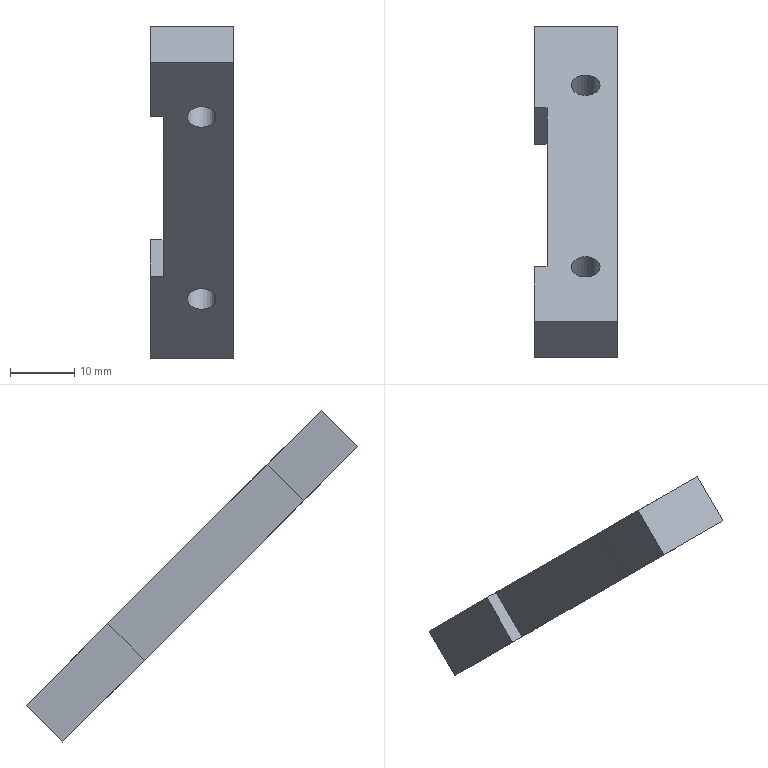Component | SolidWorks | ZL-10-05RightCoverPlate-1 | 1 solid | 14 faces | box 13 x 51.62 x 51.62 mm | volume 5946 mm3 | plane 10 | cylinder 4 | commonest cylinder face diameters 4.5 x4
build123d program:
from build123d import *

# Parameters (mm, degrees)
SKETCH1_W          = 13
SKETCH1_H          = 65
EXTRUDE1_DEPTH     = 4
SKETCH2_R          = 2.25
CUT_EXTRUDE1_DEPTH = 66.812
SKETCH3_W          = 2
SKETCH3_H          = 35
CUT_EXTRUDE2_DEPTH = 66.812


with BuildPart() as part:
    # Sketch1 → Extrude1 (new, symmetric)
    with BuildSketch(Plane.XY):
        with Locations((0, 32.5)):
            Rectangle(SKETCH1_W, SKETCH1_H)
    extrude(amount=EXTRUDE1_DEPTH, both=True)

    # Sketch2 → Cut-Extrude1 (cut, through all)
    with BuildSketch(Plane.XY.offset(4)):
        with Locations((1.5, 12)):
            Circle(SKETCH2_R)
        with Locations((1.5, 52)):
            Circle(SKETCH2_R)
    extrude(amount=-CUT_EXTRUDE1_DEPTH, mode=Mode.SUBTRACT)

    # Sketch3 → Cut-Extrude2 (cut, through all)
    with BuildSketch(Plane.XY.offset(4)):
        with Locations((-5.5, 29.5)):
            Rectangle(SKETCH3_W, SKETCH3_H)
    extrude(amount=-CUT_EXTRUDE2_DEPTH, mode=Mode.SUBTRACT)


solid = part.part

# Placed as in the assembly
solid = solid.moved(Location((56.323, 52.714, 18.077), (-45, 0, 0)))